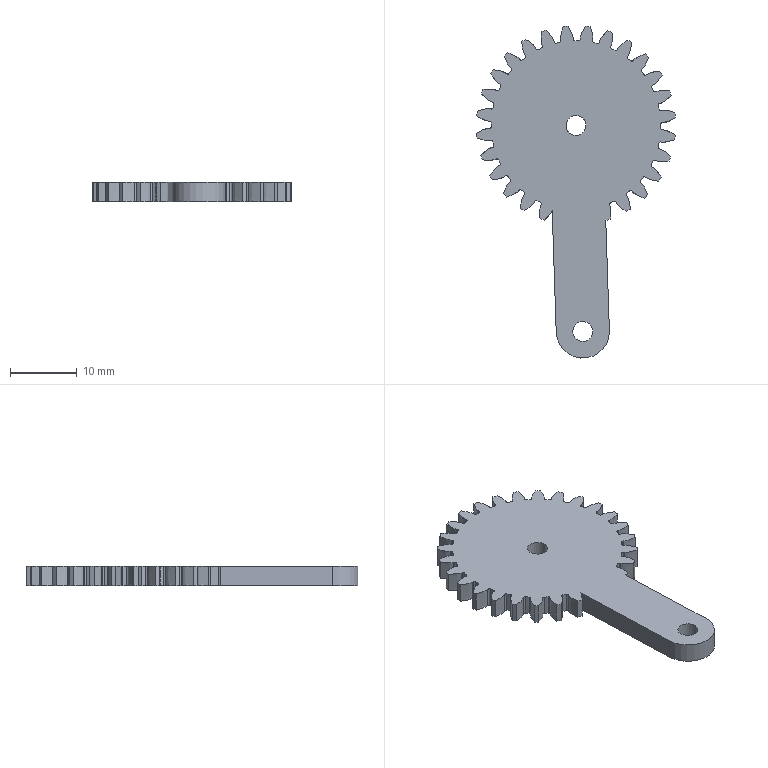Component | NX | GEAR-LINK-1_YEN | 1 solid | 210 faces | volume 2272 mm3 | cylinder 104 | plane 54 | other 52 | commonest cylinder face diameters 0.5 x50 30 x26 25.5 x25 3 x2 8 x1